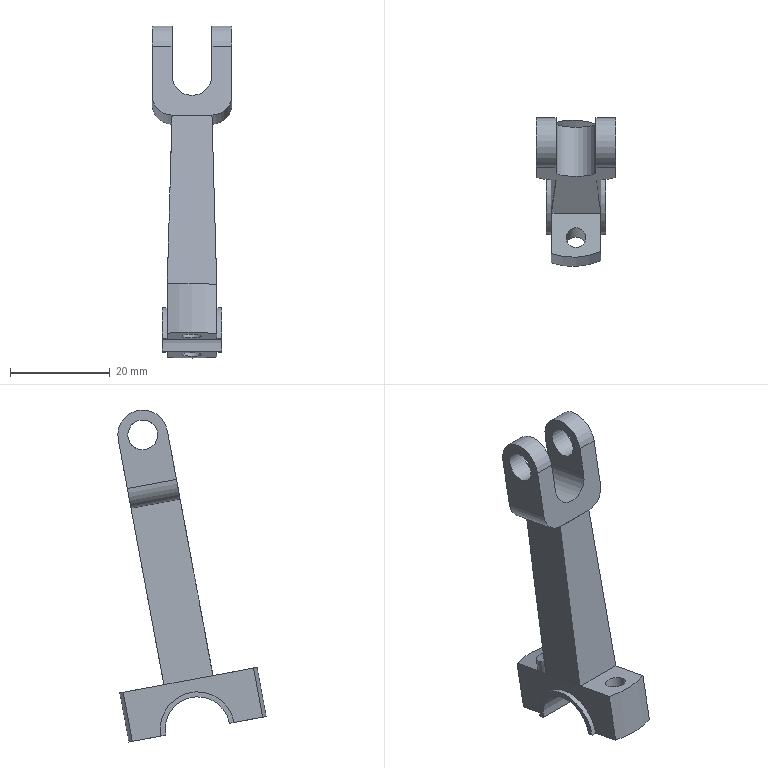Component | NX | 17A__27 | 2 solids | 32 faces | volume 6640 mm3 | plane 16 | cylinder 14 | spline 2 | commonest cylinder face diameters 8 x3 10 x2 6 x2 28 x2 4 x2 15 x2 13 x1